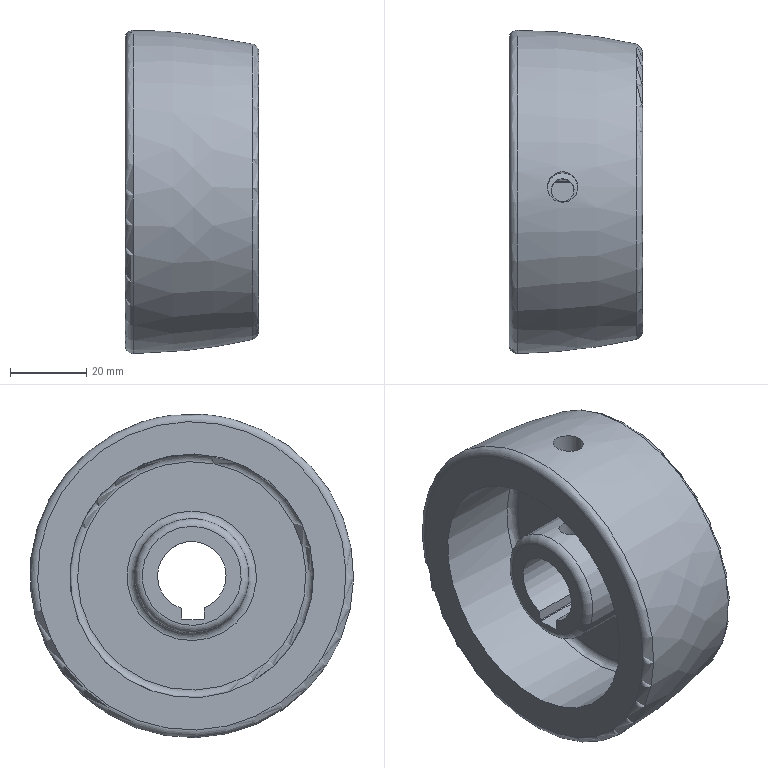Component | NX | PULLEY | 1 solid | 26 faces | volume 101287 mm3 | plane 11 | torus 7 | cylinder 7 | spline 1 | commonest cylinder face diameters 64 x2 30 x2 18 x1 8 x1 6 x1